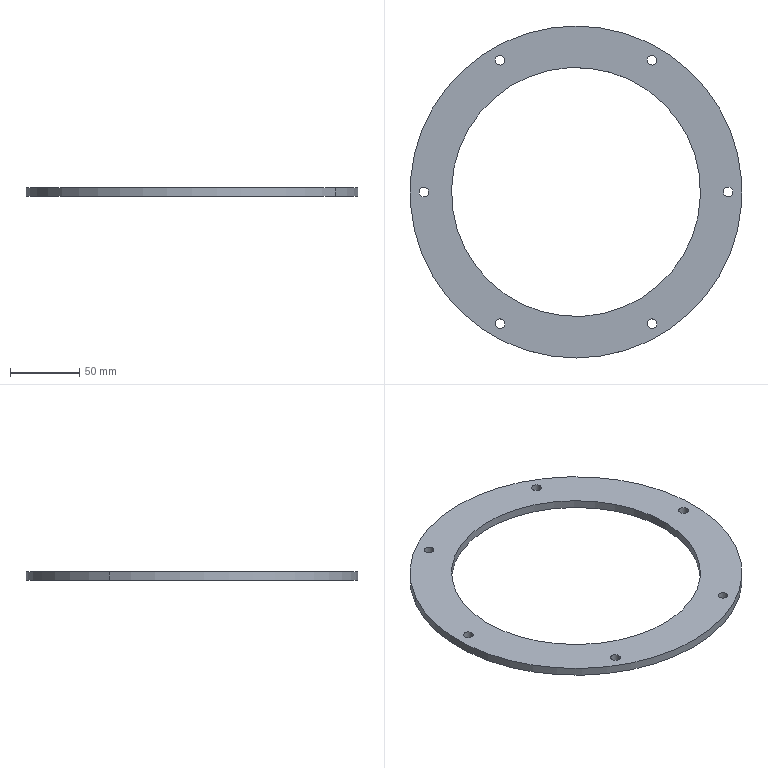Component | SolidWorks | YC1-250-02-03FrontDriveBearingSeatAssembly-1_YC1-250-02-23FrontDriveBearingSeatGland-1 | 1 solid | 18 faces | box 240 x 240 x 6 mm | volume 117367 mm3 | cylinder 16 | plane 2 | commonest cylinder face diameters 7 x12 180 x2 240 x2 | material Plain Carbon Steel
STEP:
#1=CARTESIAN_POINT('',(3.069,106.063,-17.48));
#2=VERTEX_POINT('',#1);
#3=CARTESIAN_POINT('',(-3.069,109.606,-17.48));
#4=VERTEX_POINT('',#3);
#5=CARTESIAN_POINT('',(0.,107.835,-17.48));
#6=DIRECTION('',(0.,0.,-1.));
#7=DIRECTION('',(-0.866,0.5,0.));
#8=AXIS2_PLACEMENT_3D('',#5,#6,#7);
#9=CIRCLE('',#8,3.543);
#10=EDGE_CURVE('',#2,#4,#9,.T.);
#11=ORIENTED_EDGE('',*,*,#10,.F.);
#12=CARTESIAN_POINT('',(3.069,106.063,-17.717));
#13=VERTEX_POINT('',#12);
#14=CARTESIAN_POINT('',(3.069,106.063,-17.48));
#15=DIRECTION('',(0.,0.,-1.));
#16=VECTOR('',#15,39.37);
#17=LINE('',#14,#16);
#18=EDGE_CURVE('',#2,#13,#17,.T.);
#19=ORIENTED_EDGE('',*,*,#18,.T.);
#20=CARTESIAN_POINT('',(-3.069,109.606,-17.717));
#21=VERTEX_POINT('',#20);
#22=CARTESIAN_POINT('',(0.,107.835,-17.717));
#23=DIRECTION('',(0.,0.,-1.));
#24=DIRECTION('',(-0.866,0.5,0.));
#25=AXIS2_PLACEMENT_3D('',#22,#23,#24);
#26=CIRCLE('',#25,3.543);
#27=EDGE_CURVE('',#13,#21,#26,.T.);
#28=ORIENTED_EDGE('',*,*,#27,.T.);
#29=CARTESIAN_POINT('',(-3.069,109.606,-17.48));
#30=DIRECTION('',(0.,0.,-1.));
#31=VECTOR('',#30,39.37);
#32=LINE('',#29,#31);
#33=EDGE_CURVE('',#4,#21,#32,.T.);
#34=ORIENTED_EDGE('',*,*,#33,.F.);
#35=EDGE_LOOP('',(#11,#19,#28,#34));
#36=FACE_OUTER_BOUND('',#35,.T.);
#37=CARTESIAN_POINT('',(0.,107.835,-17.48));
#38=DIRECTION('',(0.,0.,-1.));
#39=DIRECTION('',(-0.866,0.5,0.));
#40=AXIS2_PLACEMENT_3D('',#37,#38,#39);
#41=CYLINDRICAL_SURFACE('',#40,3.543);
#42=ADVANCED_FACE('',(#36),#41,.F.);
#43=CARTESIAN_POINT('',(-4.091,110.197,-17.48));
#44=VERTEX_POINT('',#43);
#45=CARTESIAN_POINT('',(4.091,105.472,-17.48));
#46=VERTEX_POINT('',#45);
#47=CARTESIAN_POINT('',(0.,107.835,-17.48));
#48=DIRECTION('',(0.,0.,-1.));
#49=DIRECTION('',(-0.866,0.5,0.));
#50=AXIS2_PLACEMENT_3D('',#47,#48,#49);
#51=CIRCLE('',#50,4.724);
#52=EDGE_CURVE('',#44,#46,#51,.T.);
#53=ORIENTED_EDGE('',*,*,#52,.T.);
#54=CARTESIAN_POINT('',(4.091,105.472,-17.717));
#55=VERTEX_POINT('',#54);
#56=CARTESIAN_POINT('',(4.091,105.472,-17.48));
#57=DIRECTION('',(0.,0.,-1.));
#58=VECTOR('',#57,39.37);
#59=LINE('',#56,#58);
#60=EDGE_CURVE('',#46,#55,#59,.T.);
#61=ORIENTED_EDGE('',*,*,#60,.T.);
#62=CARTESIAN_POINT('',(-4.091,110.197,-17.717));
#63=VERTEX_POINT('',#62);
#64=CARTESIAN_POINT('',(0.,107.835,-17.717));
#65=DIRECTION('',(0.,0.,1.));
#66=DIRECTION('',(-0.866,0.5,0.));
#67=AXIS2_PLACEMENT_3D('',#64,#65,#66);
#68=CIRCLE('',#67,4.724);
#69=EDGE_CURVE('',#55,#63,#68,.T.);
#70=ORIENTED_EDGE('',*,*,#69,.T.);
#71=CARTESIAN_POINT('',(-4.091,110.197,-17.48));
#72=DIRECTION('',(0.,0.,-1.));
#73=VECTOR('',#72,39.37);
#74=LINE('',#71,#73);
#75=EDGE_CURVE('',#44,#63,#74,.T.);
#76=ORIENTED_EDGE('',*,*,#75,.F.);
#77=EDGE_LOOP('',(#53,#61,#70,#76));
#78=FACE_OUTER_BOUND('',#77,.T.);
#79=CARTESIAN_POINT('',(0.,107.835,-17.48));
#80=DIRECTION('',(0.,0.,-1.));
#81=DIRECTION('',(-0.866,0.5,0.));
#82=AXIS2_PLACEMENT_3D('',#79,#80,#81);
#83=CYLINDRICAL_SURFACE('',#82,4.724);
#84=ADVANCED_FACE('',(#78),#83,.T.);
#85=CARTESIAN_POINT('',(-2.046,111.516,-17.717));
#86=VERTEX_POINT('',#85);
#87=CARTESIAN_POINT('',(-2.285,111.654,-17.717));
#88=VERTEX_POINT('',#87);
#89=CARTESIAN_POINT('',(-2.165,111.585,-17.717));
#90=DIRECTION('',(0.,0.,-1.));
#91=DIRECTION('',(0.866,-0.5,0.));
#92=AXIS2_PLACEMENT_3D('',#89,#90,#91);
#93=CIRCLE('',#92,0.1378);
#94=EDGE_CURVE('',#86,#88,#93,.T.);
#95=ORIENTED_EDGE('',*,*,#94,.T.);
#96=CARTESIAN_POINT('',(-2.285,111.654,-17.48));
#97=VERTEX_POINT('',#96);
#98=CARTESIAN_POINT('',(-2.285,111.654,-17.48));
#99=DIRECTION('',(0.,0.,1.));
#100=VECTOR('',#99,39.37);
#101=LINE('',#98,#100);
#102=EDGE_CURVE('',#88,#97,#101,.T.);
#103=ORIENTED_EDGE('',*,*,#102,.T.);
#104=CARTESIAN_POINT('',(-2.046,111.516,-17.48));
#105=VERTEX_POINT('',#104);
#106=CARTESIAN_POINT('',(-2.165,111.585,-17.48));
#107=DIRECTION('',(0.,0.,-1.));
#108=DIRECTION('',(0.866,-0.5,0.));
#109=AXIS2_PLACEMENT_3D('',#106,#107,#108);
#110=CIRCLE('',#109,0.1378);
#111=EDGE_CURVE('',#105,#97,#110,.T.);
#112=ORIENTED_EDGE('',*,*,#111,.F.);
#113=CARTESIAN_POINT('',(-2.046,111.516,-17.48));
#114=DIRECTION('',(0.,0.,1.));
#115=VECTOR('',#114,39.37);
#116=LINE('',#113,#115);
#117=EDGE_CURVE('',#86,#105,#116,.T.);
#118=ORIENTED_EDGE('',*,*,#117,.F.);
#119=EDGE_LOOP('',(#95,#103,#112,#118));
#120=FACE_OUTER_BOUND('',#119,.T.);
#121=CARTESIAN_POINT('',(-2.165,111.585,-17.48));
#122=DIRECTION('',(0.,0.,1.));
#123=DIRECTION('',(0.866,-0.5,0.));
#124=AXIS2_PLACEMENT_3D('',#121,#122,#123);
#125=CYLINDRICAL_SURFACE('',#124,0.1378);
#126=ADVANCED_FACE('',(#120),#125,.F.);
#127=CARTESIAN_POINT('',(-4.211,107.766,-17.717));
#128=VERTEX_POINT('',#127);
#129=CARTESIAN_POINT('',(-4.45,107.904,-17.717));
#130=VERTEX_POINT('',#129);
#131=CARTESIAN_POINT('',(-4.331,107.835,-17.717));
#132=DIRECTION('',(0.,0.,-1.));
#133=DIRECTION('',(0.866,-0.5,0.));
#134=AXIS2_PLACEMENT_3D('',#131,#132,#133);
#135=CIRCLE('',#134,0.1378);
#136=EDGE_CURVE('',#128,#130,#135,.T.);
#137=ORIENTED_EDGE('',*,*,#136,.T.);
#138=CARTESIAN_POINT('',(-4.45,107.904,-17.48));
#139=VERTEX_POINT('',#138);
#140=CARTESIAN_POINT('',(-4.45,107.904,-17.48));
#141=DIRECTION('',(0.,0.,1.));
#142=VECTOR('',#141,39.37);
#143=LINE('',#140,#142);
#144=EDGE_CURVE('',#130,#139,#143,.T.);
#145=ORIENTED_EDGE('',*,*,#144,.T.);
#146=CARTESIAN_POINT('',(-4.211,107.766,-17.48));
#147=VERTEX_POINT('',#146);
#148=CARTESIAN_POINT('',(-4.331,107.835,-17.48));
#149=DIRECTION('',(0.,0.,-1.));
#150=DIRECTION('',(0.866,-0.5,0.));
#151=AXIS2_PLACEMENT_3D('',#148,#149,#150);
#152=CIRCLE('',#151,0.1378);
#153=EDGE_CURVE('',#147,#139,#152,.T.);
#154=ORIENTED_EDGE('',*,*,#153,.F.);
#155=CARTESIAN_POINT('',(-4.211,107.766,-17.48));
#156=DIRECTION('',(0.,0.,1.));
#157=VECTOR('',#156,39.37);
#158=LINE('',#155,#157);
#159=EDGE_CURVE('',#128,#147,#158,.T.);
#160=ORIENTED_EDGE('',*,*,#159,.F.);
#161=EDGE_LOOP('',(#137,#145,#154,#160));
#162=FACE_OUTER_BOUND('',#161,.T.);
#163=CARTESIAN_POINT('',(-4.331,107.835,-17.48));
#164=DIRECTION('',(0.,0.,1.));
#165=DIRECTION('',(0.866,-0.5,0.));
#166=AXIS2_PLACEMENT_3D('',#163,#164,#165);
#167=CYLINDRICAL_SURFACE('',#166,0.1378);
#168=ADVANCED_FACE('',(#162),#167,.F.);
#169=CARTESIAN_POINT('',(-2.046,104.015,-17.717));
#170=VERTEX_POINT('',#169);
#171=CARTESIAN_POINT('',(-2.285,104.153,-17.717));
#172=VERTEX_POINT('',#171);
#173=CARTESIAN_POINT('',(-2.165,104.084,-17.717));
#174=DIRECTION('',(0.,0.,-1.));
#175=DIRECTION('',(0.866,-0.5,0.));
#176=AXIS2_PLACEMENT_3D('',#173,#174,#175);
#177=CIRCLE('',#176,0.1378);
#178=EDGE_CURVE('',#170,#172,#177,.T.);
#179=ORIENTED_EDGE('',*,*,#178,.T.);
#180=CARTESIAN_POINT('',(-2.285,104.153,-17.48));
#181=VERTEX_POINT('',#180);
#182=CARTESIAN_POINT('',(-2.285,104.153,-17.48));
#183=DIRECTION('',(0.,0.,1.));
#184=VECTOR('',#183,39.37);
#185=LINE('',#182,#184);
#186=EDGE_CURVE('',#172,#181,#185,.T.);
#187=ORIENTED_EDGE('',*,*,#186,.T.);
#188=CARTESIAN_POINT('',(-2.046,104.015,-17.48));
#189=VERTEX_POINT('',#188);
#190=CARTESIAN_POINT('',(-2.165,104.084,-17.48));
#191=DIRECTION('',(0.,0.,-1.));
#192=DIRECTION('',(0.866,-0.5,0.));
#193=AXIS2_PLACEMENT_3D('',#190,#191,#192);
#194=CIRCLE('',#193,0.1378);
#195=EDGE_CURVE('',#189,#181,#194,.T.);
#196=ORIENTED_EDGE('',*,*,#195,.F.);
#197=CARTESIAN_POINT('',(-2.046,104.015,-17.48));
#198=DIRECTION('',(0.,0.,1.));
#199=VECTOR('',#198,39.37);
#200=LINE('',#197,#199);
#201=EDGE_CURVE('',#170,#189,#200,.T.);
#202=ORIENTED_EDGE('',*,*,#201,.F.);
#203=EDGE_LOOP('',(#179,#187,#196,#202));
#204=FACE_OUTER_BOUND('',#203,.T.);
#205=CARTESIAN_POINT('',(-2.165,104.084,-17.48));
#206=DIRECTION('',(0.,0.,1.));
#207=DIRECTION('',(0.866,-0.5,0.));
#208=AXIS2_PLACEMENT_3D('',#205,#206,#207);
#209=CYLINDRICAL_SURFACE('',#208,0.1378);
#210=ADVANCED_FACE('',(#204),#209,.F.);
#211=CARTESIAN_POINT('',(2.285,104.015,-17.717));
#212=VERTEX_POINT('',#211);
#213=CARTESIAN_POINT('',(2.046,104.153,-17.717));
#214=VERTEX_POINT('',#213);
#215=CARTESIAN_POINT('',(2.165,104.084,-17.717));
#216=DIRECTION('',(0.,0.,-1.));
#217=DIRECTION('',(0.866,-0.5,0.));
#218=AXIS2_PLACEMENT_3D('',#215,#216,#217);
#219=CIRCLE('',#218,0.1378);
#220=EDGE_CURVE('',#212,#214,#219,.T.);
#221=ORIENTED_EDGE('',*,*,#220,.T.);
#222=CARTESIAN_POINT('',(2.046,104.153,-17.48));
#223=VERTEX_POINT('',#222);
#224=CARTESIAN_POINT('',(2.046,104.153,-17.48));
#225=DIRECTION('',(0.,0.,1.));
#226=VECTOR('',#225,39.37);
#227=LINE('',#224,#226);
#228=EDGE_CURVE('',#214,#223,#227,.T.);
#229=ORIENTED_EDGE('',*,*,#228,.T.);
#230=CARTESIAN_POINT('',(2.285,104.015,-17.48));
#231=VERTEX_POINT('',#230);
#232=CARTESIAN_POINT('',(2.165,104.084,-17.48));
#233=DIRECTION('',(0.,0.,-1.));
#234=DIRECTION('',(0.866,-0.5,0.));
#235=AXIS2_PLACEMENT_3D('',#232,#233,#234);
#236=CIRCLE('',#235,0.1378);
#237=EDGE_CURVE('',#231,#223,#236,.T.);
#238=ORIENTED_EDGE('',*,*,#237,.F.);
#239=CARTESIAN_POINT('',(2.285,104.015,-17.48));
#240=DIRECTION('',(0.,0.,1.));
#241=VECTOR('',#240,39.37);
#242=LINE('',#239,#241);
#243=EDGE_CURVE('',#212,#231,#242,.T.);
#244=ORIENTED_EDGE('',*,*,#243,.F.);
#245=EDGE_LOOP('',(#221,#229,#238,#244));
#246=FACE_OUTER_BOUND('',#245,.T.);
#247=CARTESIAN_POINT('',(2.165,104.084,-17.48));
#248=DIRECTION('',(0.,0.,1.));
#249=DIRECTION('',(0.866,-0.5,0.));
#250=AXIS2_PLACEMENT_3D('',#247,#248,#249);
#251=CYLINDRICAL_SURFACE('',#250,0.1378);
#252=ADVANCED_FACE('',(#246),#251,.F.);
#253=CARTESIAN_POINT('',(4.45,107.766,-17.717));
#254=VERTEX_POINT('',#253);
#255=CARTESIAN_POINT('',(4.211,107.904,-17.717));
#256=VERTEX_POINT('',#255);
#257=CARTESIAN_POINT('',(4.331,107.835,-17.717));
#258=DIRECTION('',(0.,0.,-1.));
#259=DIRECTION('',(0.866,-0.5,0.));
#260=AXIS2_PLACEMENT_3D('',#257,#258,#259);
#261=CIRCLE('',#260,0.1378);
#262=EDGE_CURVE('',#254,#256,#261,.T.);
#263=ORIENTED_EDGE('',*,*,#262,.T.);
#264=CARTESIAN_POINT('',(4.211,107.904,-17.48));
#265=VERTEX_POINT('',#264);
#266=CARTESIAN_POINT('',(4.211,107.904,-17.48));
#267=DIRECTION('',(0.,0.,1.));
#268=VECTOR('',#267,39.37);
#269=LINE('',#266,#268);
#270=EDGE_CURVE('',#256,#265,#269,.T.);
#271=ORIENTED_EDGE('',*,*,#270,.T.);
#272=CARTESIAN_POINT('',(4.45,107.766,-17.48));
#273=VERTEX_POINT('',#272);
#274=CARTESIAN_POINT('',(4.331,107.835,-17.48));
#275=DIRECTION('',(0.,0.,-1.));
#276=DIRECTION('',(0.866,-0.5,0.));
#277=AXIS2_PLACEMENT_3D('',#274,#275,#276);
#278=CIRCLE('',#277,0.1378);
#279=EDGE_CURVE('',#273,#265,#278,.T.);
#280=ORIENTED_EDGE('',*,*,#279,.F.);
#281=CARTESIAN_POINT('',(4.45,107.766,-17.48));
#282=DIRECTION('',(0.,0.,1.));
#283=VECTOR('',#282,39.37);
#284=LINE('',#281,#283);
#285=EDGE_CURVE('',#254,#273,#284,.T.);
#286=ORIENTED_EDGE('',*,*,#285,.F.);
#287=EDGE_LOOP('',(#263,#271,#280,#286));
#288=FACE_OUTER_BOUND('',#287,.T.);
#289=CARTESIAN_POINT('',(4.331,107.835,-17.48));
#290=DIRECTION('',(0.,0.,1.));
#291=DIRECTION('',(0.866,-0.5,0.));
#292=AXIS2_PLACEMENT_3D('',#289,#290,#291);
#293=CYLINDRICAL_SURFACE('',#292,0.1378);
#294=ADVANCED_FACE('',(#288),#293,.F.);
#295=CARTESIAN_POINT('',(2.285,111.516,-17.717));
#296=VERTEX_POINT('',#295);
#297=CARTESIAN_POINT('',(2.046,111.654,-17.717));
#298=VERTEX_POINT('',#297);
#299=CARTESIAN_POINT('',(2.165,111.585,-17.717));
#300=DIRECTION('',(0.,0.,-1.));
#301=DIRECTION('',(0.866,-0.5,0.));
#302=AXIS2_PLACEMENT_3D('',#299,#300,#301);
#303=CIRCLE('',#302,0.1378);
#304=EDGE_CURVE('',#296,#298,#303,.T.);
#305=ORIENTED_EDGE('',*,*,#304,.T.);
#306=CARTESIAN_POINT('',(2.046,111.654,-17.48));
#307=VERTEX_POINT('',#306);
#308=CARTESIAN_POINT('',(2.046,111.654,-17.48));
#309=DIRECTION('',(0.,0.,1.));
#310=VECTOR('',#309,39.37);
#311=LINE('',#308,#310);
#312=EDGE_CURVE('',#298,#307,#311,.T.);
#313=ORIENTED_EDGE('',*,*,#312,.T.);
#314=CARTESIAN_POINT('',(2.285,111.516,-17.48));
#315=VERTEX_POINT('',#314);
#316=CARTESIAN_POINT('',(2.165,111.585,-17.48));
#317=DIRECTION('',(0.,0.,-1.));
#318=DIRECTION('',(0.866,-0.5,0.));
#319=AXIS2_PLACEMENT_3D('',#316,#317,#318);
#320=CIRCLE('',#319,0.1378);
#321=EDGE_CURVE('',#315,#307,#320,.T.);
#322=ORIENTED_EDGE('',*,*,#321,.F.);
#323=CARTESIAN_POINT('',(2.285,111.516,-17.48));
#324=DIRECTION('',(0.,0.,1.));
#325=VECTOR('',#324,39.37);
#326=LINE('',#323,#325);
#327=EDGE_CURVE('',#296,#315,#326,.T.);
#328=ORIENTED_EDGE('',*,*,#327,.F.);
#329=EDGE_LOOP('',(#305,#313,#322,#328));
#330=FACE_OUTER_BOUND('',#329,.T.);
#331=CARTESIAN_POINT('',(2.165,111.585,-17.48));
#332=DIRECTION('',(0.,0.,1.));
#333=DIRECTION('',(0.866,-0.5,0.));
#334=AXIS2_PLACEMENT_3D('',#331,#332,#333);
#335=CYLINDRICAL_SURFACE('',#334,0.1378);
#336=ADVANCED_FACE('',(#330),#335,.F.);
#337=CARTESIAN_POINT('',(0.,107.835,-17.717));
#338=DIRECTION('',(0.,0.,-1.));
#339=DIRECTION('',(-0.866,0.5,0.));
#340=AXIS2_PLACEMENT_3D('',#337,#338,#339);
#341=CIRCLE('',#340,3.543);
#342=EDGE_CURVE('',#21,#13,#341,.T.);
#343=ORIENTED_EDGE('',*,*,#342,.F.);
#344=ORIENTED_EDGE('',*,*,#27,.F.);
#345=EDGE_LOOP('',(#343,#344));
#346=FACE_BOUND('',#345,.T.);
#347=CARTESIAN_POINT('',(0.,107.835,-17.717));
#348=DIRECTION('',(0.,0.,1.));
#349=DIRECTION('',(-0.866,0.5,0.));
#350=AXIS2_PLACEMENT_3D('',#347,#348,#349);
#351=CIRCLE('',#350,4.724);
#352=EDGE_CURVE('',#63,#55,#351,.T.);
#353=ORIENTED_EDGE('',*,*,#352,.F.);
#354=ORIENTED_EDGE('',*,*,#69,.F.);
#355=EDGE_LOOP('',(#353,#354));
#356=FACE_OUTER_BOUND('',#355,.T.);
#357=ORIENTED_EDGE('',*,*,#94,.F.);
#358=CARTESIAN_POINT('',(-2.165,111.585,-17.717));
#359=DIRECTION('',(0.,0.,-1.));
#360=DIRECTION('',(0.866,-0.5,0.));
#361=AXIS2_PLACEMENT_3D('',#358,#359,#360);
#362=CIRCLE('',#361,0.1378);
#363=EDGE_CURVE('',#88,#86,#362,.T.);
#364=ORIENTED_EDGE('',*,*,#363,.F.);
#365=EDGE_LOOP('',(#357,#364));
#366=FACE_BOUND('',#365,.T.);
#367=ORIENTED_EDGE('',*,*,#136,.F.);
#368=CARTESIAN_POINT('',(-4.331,107.835,-17.717));
#369=DIRECTION('',(0.,0.,-1.));
#370=DIRECTION('',(0.866,-0.5,0.));
#371=AXIS2_PLACEMENT_3D('',#368,#369,#370);
#372=CIRCLE('',#371,0.1378);
#373=EDGE_CURVE('',#130,#128,#372,.T.);
#374=ORIENTED_EDGE('',*,*,#373,.F.);
#375=EDGE_LOOP('',(#367,#374));
#376=FACE_BOUND('',#375,.T.);
#377=ORIENTED_EDGE('',*,*,#178,.F.);
#378=CARTESIAN_POINT('',(-2.165,104.084,-17.717));
#379=DIRECTION('',(0.,0.,-1.));
#380=DIRECTION('',(0.866,-0.5,0.));
#381=AXIS2_PLACEMENT_3D('',#378,#379,#380);
#382=CIRCLE('',#381,0.1378);
#383=EDGE_CURVE('',#172,#170,#382,.T.);
#384=ORIENTED_EDGE('',*,*,#383,.F.);
#385=EDGE_LOOP('',(#377,#384));
#386=FACE_BOUND('',#385,.T.);
#387=ORIENTED_EDGE('',*,*,#220,.F.);
#388=CARTESIAN_POINT('',(2.165,104.084,-17.717));
#389=DIRECTION('',(0.,0.,-1.));
#390=DIRECTION('',(0.866,-0.5,0.));
#391=AXIS2_PLACEMENT_3D('',#388,#389,#390);
#392=CIRCLE('',#391,0.1378);
#393=EDGE_CURVE('',#214,#212,#392,.T.);
#394=ORIENTED_EDGE('',*,*,#393,.F.);
#395=EDGE_LOOP('',(#387,#394));
#396=FACE_BOUND('',#395,.T.);
#397=ORIENTED_EDGE('',*,*,#262,.F.);
#398=CARTESIAN_POINT('',(4.331,107.835,-17.717));
#399=DIRECTION('',(0.,0.,-1.));
#400=DIRECTION('',(0.866,-0.5,0.));
#401=AXIS2_PLACEMENT_3D('',#398,#399,#400);
#402=CIRCLE('',#401,0.1378);
#403=EDGE_CURVE('',#256,#254,#402,.T.);
#404=ORIENTED_EDGE('',*,*,#403,.F.);
#405=EDGE_LOOP('',(#397,#404));
#406=FACE_BOUND('',#405,.T.);
#407=ORIENTED_EDGE('',*,*,#304,.F.);
#408=CARTESIAN_POINT('',(2.165,111.585,-17.717));
#409=DIRECTION('',(0.,0.,-1.));
#410=DIRECTION('',(0.866,-0.5,0.));
#411=AXIS2_PLACEMENT_3D('',#408,#409,#410);
#412=CIRCLE('',#411,0.1378);
#413=EDGE_CURVE('',#298,#296,#412,.T.);
#414=ORIENTED_EDGE('',*,*,#413,.F.);
#415=EDGE_LOOP('',(#407,#414));
#416=FACE_BOUND('',#415,.T.);
#417=CARTESIAN_POINT('',(0.,107.835,-17.717));
#418=DIRECTION('',(0.,0.,1.));
#419=DIRECTION('',(0.866,-0.5,0.));
#420=AXIS2_PLACEMENT_3D('',#417,#418,#419);
#421=PLANE('',#420);
#422=ADVANCED_FACE('',(#346,#356,#366,#376,#386,#396,#406,#416),#421,.F.);
#423=ORIENTED_EDGE('',*,*,#18,.F.);
#424=CARTESIAN_POINT('',(0.,107.835,-17.48));
#425=DIRECTION('',(0.,0.,-1.));
#426=DIRECTION('',(-0.866,0.5,0.));
#427=AXIS2_PLACEMENT_3D('',#424,#425,#426);
#428=CIRCLE('',#427,3.543);
#429=EDGE_CURVE('',#4,#2,#428,.T.);
#430=ORIENTED_EDGE('',*,*,#429,.F.);
#431=ORIENTED_EDGE('',*,*,#33,.T.);
#432=ORIENTED_EDGE('',*,*,#342,.T.);
#433=EDGE_LOOP('',(#423,#430,#431,#432));
#434=FACE_OUTER_BOUND('',#433,.T.);
#435=CARTESIAN_POINT('',(0.,107.835,-17.48));
#436=DIRECTION('',(0.,0.,-1.));
#437=DIRECTION('',(-0.866,0.5,0.));
#438=AXIS2_PLACEMENT_3D('',#435,#436,#437);
#439=CYLINDRICAL_SURFACE('',#438,3.543);
#440=ADVANCED_FACE('',(#434),#439,.F.);
#441=ORIENTED_EDGE('',*,*,#60,.F.);
#442=CARTESIAN_POINT('',(0.,107.835,-17.48));
#443=DIRECTION('',(0.,0.,-1.));
#444=DIRECTION('',(-0.866,0.5,0.));
#445=AXIS2_PLACEMENT_3D('',#442,#443,#444);
#446=CIRCLE('',#445,4.724);
#447=EDGE_CURVE('',#46,#44,#446,.T.);
#448=ORIENTED_EDGE('',*,*,#447,.T.);
#449=ORIENTED_EDGE('',*,*,#75,.T.);
#450=ORIENTED_EDGE('',*,*,#352,.T.);
#451=EDGE_LOOP('',(#441,#448,#449,#450));
#452=FACE_OUTER_BOUND('',#451,.T.);
#453=CARTESIAN_POINT('',(0.,107.835,-17.48));
#454=DIRECTION('',(0.,0.,-1.));
#455=DIRECTION('',(-0.866,0.5,0.));
#456=AXIS2_PLACEMENT_3D('',#453,#454,#455);
#457=CYLINDRICAL_SURFACE('',#456,4.724);
#458=ADVANCED_FACE('',(#452),#457,.T.);
#459=ORIENTED_EDGE('',*,*,#102,.F.);
#460=ORIENTED_EDGE('',*,*,#363,.T.);
#461=ORIENTED_EDGE('',*,*,#117,.T.);
#462=CARTESIAN_POINT('',(-2.165,111.585,-17.48));
#463=DIRECTION('',(0.,0.,-1.));
#464=DIRECTION('',(0.866,-0.5,0.));
#465=AXIS2_PLACEMENT_3D('',#462,#463,#464);
#466=CIRCLE('',#465,0.1378);
#467=EDGE_CURVE('',#97,#105,#466,.T.);
#468=ORIENTED_EDGE('',*,*,#467,.F.);
#469=EDGE_LOOP('',(#459,#460,#461,#468));
#470=FACE_OUTER_BOUND('',#469,.T.);
#471=CARTESIAN_POINT('',(-2.165,111.585,-17.48));
#472=DIRECTION('',(0.,0.,1.));
#473=DIRECTION('',(0.866,-0.5,0.));
#474=AXIS2_PLACEMENT_3D('',#471,#472,#473);
#475=CYLINDRICAL_SURFACE('',#474,0.1378);
#476=ADVANCED_FACE('',(#470),#475,.F.);
#477=ORIENTED_EDGE('',*,*,#144,.F.);
#478=ORIENTED_EDGE('',*,*,#373,.T.);
#479=ORIENTED_EDGE('',*,*,#159,.T.);
#480=CARTESIAN_POINT('',(-4.331,107.835,-17.48));
#481=DIRECTION('',(0.,0.,-1.));
#482=DIRECTION('',(0.866,-0.5,0.));
#483=AXIS2_PLACEMENT_3D('',#480,#481,#482);
#484=CIRCLE('',#483,0.1378);
#485=EDGE_CURVE('',#139,#147,#484,.T.);
#486=ORIENTED_EDGE('',*,*,#485,.F.);
#487=EDGE_LOOP('',(#477,#478,#479,#486));
#488=FACE_OUTER_BOUND('',#487,.T.);
#489=CARTESIAN_POINT('',(-4.331,107.835,-17.48));
#490=DIRECTION('',(0.,0.,1.));
#491=DIRECTION('',(0.866,-0.5,0.));
#492=AXIS2_PLACEMENT_3D('',#489,#490,#491);
#493=CYLINDRICAL_SURFACE('',#492,0.1378);
#494=ADVANCED_FACE('',(#488),#493,.F.);
#495=ORIENTED_EDGE('',*,*,#186,.F.);
#496=ORIENTED_EDGE('',*,*,#383,.T.);
#497=ORIENTED_EDGE('',*,*,#201,.T.);
#498=CARTESIAN_POINT('',(-2.165,104.084,-17.48));
#499=DIRECTION('',(0.,0.,-1.));
#500=DIRECTION('',(0.866,-0.5,0.));
#501=AXIS2_PLACEMENT_3D('',#498,#499,#500);
#502=CIRCLE('',#501,0.1378);
#503=EDGE_CURVE('',#181,#189,#502,.T.);
#504=ORIENTED_EDGE('',*,*,#503,.F.);
#505=EDGE_LOOP('',(#495,#496,#497,#504));
#506=FACE_OUTER_BOUND('',#505,.T.);
#507=CARTESIAN_POINT('',(-2.165,104.084,-17.48));
#508=DIRECTION('',(0.,0.,1.));
#509=DIRECTION('',(0.866,-0.5,0.));
#510=AXIS2_PLACEMENT_3D('',#507,#508,#509);
#511=CYLINDRICAL_SURFACE('',#510,0.1378);
#512=ADVANCED_FACE('',(#506),#511,.F.);
#513=ORIENTED_EDGE('',*,*,#228,.F.);
#514=ORIENTED_EDGE('',*,*,#393,.T.);
#515=ORIENTED_EDGE('',*,*,#243,.T.);
#516=CARTESIAN_POINT('',(2.165,104.084,-17.48));
#517=DIRECTION('',(0.,0.,-1.));
#518=DIRECTION('',(0.866,-0.5,0.));
#519=AXIS2_PLACEMENT_3D('',#516,#517,#518);
#520=CIRCLE('',#519,0.1378);
#521=EDGE_CURVE('',#223,#231,#520,.T.);
#522=ORIENTED_EDGE('',*,*,#521,.F.);
#523=EDGE_LOOP('',(#513,#514,#515,#522));
#524=FACE_OUTER_BOUND('',#523,.T.);
#525=CARTESIAN_POINT('',(2.165,104.084,-17.48));
#526=DIRECTION('',(0.,0.,1.));
#527=DIRECTION('',(0.866,-0.5,0.));
#528=AXIS2_PLACEMENT_3D('',#525,#526,#527);
#529=CYLINDRICAL_SURFACE('',#528,0.1378);
#530=ADVANCED_FACE('',(#524),#529,.F.);
#531=ORIENTED_EDGE('',*,*,#270,.F.);
#532=ORIENTED_EDGE('',*,*,#403,.T.);
#533=ORIENTED_EDGE('',*,*,#285,.T.);
#534=CARTESIAN_POINT('',(4.331,107.835,-17.48));
#535=DIRECTION('',(0.,0.,-1.));
#536=DIRECTION('',(0.866,-0.5,0.));
#537=AXIS2_PLACEMENT_3D('',#534,#535,#536);
#538=CIRCLE('',#537,0.1378);
#539=EDGE_CURVE('',#265,#273,#538,.T.);
#540=ORIENTED_EDGE('',*,*,#539,.F.);
#541=EDGE_LOOP('',(#531,#532,#533,#540));
#542=FACE_OUTER_BOUND('',#541,.T.);
#543=CARTESIAN_POINT('',(4.331,107.835,-17.48));
#544=DIRECTION('',(0.,0.,1.));
#545=DIRECTION('',(0.866,-0.5,0.));
#546=AXIS2_PLACEMENT_3D('',#543,#544,#545);
#547=CYLINDRICAL_SURFACE('',#546,0.1378);
#548=ADVANCED_FACE('',(#542),#547,.F.);
#549=ORIENTED_EDGE('',*,*,#312,.F.);
#550=ORIENTED_EDGE('',*,*,#413,.T.);
#551=ORIENTED_EDGE('',*,*,#327,.T.);
#552=CARTESIAN_POINT('',(2.165,111.585,-17.48));
#553=DIRECTION('',(0.,0.,-1.));
#554=DIRECTION('',(0.866,-0.5,0.));
#555=AXIS2_PLACEMENT_3D('',#552,#553,#554);
#556=CIRCLE('',#555,0.1378);
#557=EDGE_CURVE('',#307,#315,#556,.T.);
#558=ORIENTED_EDGE('',*,*,#557,.F.);
#559=EDGE_LOOP('',(#549,#550,#551,#558));
#560=FACE_OUTER_BOUND('',#559,.T.);
#561=CARTESIAN_POINT('',(2.165,111.585,-17.48));
#562=DIRECTION('',(0.,0.,1.));
#563=DIRECTION('',(0.866,-0.5,0.));
#564=AXIS2_PLACEMENT_3D('',#561,#562,#563);
#565=CYLINDRICAL_SURFACE('',#564,0.1378);
#566=ADVANCED_FACE('',(#560),#565,.F.);
#567=ORIENTED_EDGE('',*,*,#429,.T.);
#568=ORIENTED_EDGE('',*,*,#10,.T.);
#569=EDGE_LOOP('',(#567,#568));
#570=FACE_BOUND('',#569,.T.);
#571=ORIENTED_EDGE('',*,*,#52,.F.);
#572=ORIENTED_EDGE('',*,*,#447,.F.);
#573=EDGE_LOOP('',(#571,#572));
#574=FACE_OUTER_BOUND('',#573,.T.);
#575=ORIENTED_EDGE('',*,*,#111,.T.);
#576=ORIENTED_EDGE('',*,*,#467,.T.);
#577=EDGE_LOOP('',(#575,#576));
#578=FACE_BOUND('',#577,.T.);
#579=ORIENTED_EDGE('',*,*,#153,.T.);
#580=ORIENTED_EDGE('',*,*,#485,.T.);
#581=EDGE_LOOP('',(#579,#580));
#582=FACE_BOUND('',#581,.T.);
#583=ORIENTED_EDGE('',*,*,#195,.T.);
#584=ORIENTED_EDGE('',*,*,#503,.T.);
#585=EDGE_LOOP('',(#583,#584));
#586=FACE_BOUND('',#585,.T.);
#587=ORIENTED_EDGE('',*,*,#237,.T.);
#588=ORIENTED_EDGE('',*,*,#521,.T.);
#589=EDGE_LOOP('',(#587,#588));
#590=FACE_BOUND('',#589,.T.);
#591=ORIENTED_EDGE('',*,*,#279,.T.);
#592=ORIENTED_EDGE('',*,*,#539,.T.);
#593=EDGE_LOOP('',(#591,#592));
#594=FACE_BOUND('',#593,.T.);
#595=ORIENTED_EDGE('',*,*,#321,.T.);
#596=ORIENTED_EDGE('',*,*,#557,.T.);
#597=EDGE_LOOP('',(#595,#596));
#598=FACE_BOUND('',#597,.T.);
#599=CARTESIAN_POINT('',(0.,107.835,-17.48));
#600=DIRECTION('',(0.,0.,1.));
#601=DIRECTION('',(0.866,-0.5,0.));
#602=AXIS2_PLACEMENT_3D('',#599,#600,#601);
#603=PLANE('',#602);
#604=ADVANCED_FACE('',(#570,#574,#578,#582,#586,#590,#594,#598),#603,.T.);
#605=CLOSED_SHELL('',(#42,#84,#126,#168,#210,#252,#294,#336,#422,#440,#458,#476,#494,#512,#530,#548,#566,#604));
#606=MANIFOLD_SOLID_BREP('',#605);
#607=CARTESIAN_POINT('',(0.,0.,0.));
#608=DIRECTION('',(0.,0.,1.));
#609=DIRECTION('',(1.,0.,0.));
#610=AXIS2_PLACEMENT_3D('',#607,#608,#609);
#611=(LENGTH_UNIT()NAMED_UNIT(*)SI_UNIT($,.METRE.));
#612=LENGTH_MEASURE_WITH_UNIT(LENGTH_MEASURE(0.0254),#611);
#613=DIMENSIONAL_EXPONENTS(1.,0.,0.,0.,0.,0.,0.);
#614=(CONVERSION_BASED_UNIT('',#612)LENGTH_UNIT()NAMED_UNIT(#613));
#615=UNCERTAINTY_MEASURE_WITH_UNIT(LENGTH_MEASURE(0.00001),#614,'','');
#616=(NAMED_UNIT(*)PLANE_ANGLE_UNIT()SI_UNIT($,.RADIAN.));
#617=(NAMED_UNIT(*)SI_UNIT($,.STERADIAN.)SOLID_ANGLE_UNIT());
#618=(GEOMETRIC_REPRESENTATION_CONTEXT(3)GLOBAL_UNCERTAINTY_ASSIGNED_CONTEXT((#615))GLOBAL_UNIT_ASSIGNED_CONTEXT((#614,#616,#617))REPRESENTATION_CONTEXT('',''));
#619=ADVANCED_BREP_SHAPE_REPRESENTATION('',(#606,#610),#618);
#620=COLOUR_RGB('',0.7922,0.8196,0.9333);
#621=FILL_AREA_STYLE_COLOUR('',#620);
#622=FILL_AREA_STYLE('',(#621));
#623=SURFACE_STYLE_FILL_AREA(#622);
#624=SURFACE_SIDE_STYLE('',(#623));
#625=SURFACE_STYLE_USAGE(.BOTH.,#624);
#626=PRESENTATION_STYLE_ASSIGNMENT((#625));
#627=STYLED_ITEM('',(#626),#606);
#628=PRESENTATION_LAYER_ASSIGNMENT('','',(#627));
#629=(LENGTH_UNIT()NAMED_UNIT(*)SI_UNIT($,.METRE.));
#630=LENGTH_MEASURE_WITH_UNIT(LENGTH_MEASURE(0.0254),#629);
#631=DIMENSIONAL_EXPONENTS(1.,0.,0.,0.,0.,0.,0.);
#632=(CONVERSION_BASED_UNIT('',#630)LENGTH_UNIT()NAMED_UNIT(#631));
#633=UNCERTAINTY_MEASURE_WITH_UNIT(LENGTH_MEASURE(0.00001),#632,'','');
#634=(NAMED_UNIT(*)PLANE_ANGLE_UNIT()SI_UNIT($,.RADIAN.));
#635=(NAMED_UNIT(*)SI_UNIT($,.STERADIAN.)SOLID_ANGLE_UNIT());
#636=(GEOMETRIC_REPRESENTATION_CONTEXT(3)GLOBAL_UNCERTAINTY_ASSIGNED_CONTEXT((#633))GLOBAL_UNIT_ASSIGNED_CONTEXT((#632,#634,#635))REPRESENTATION_CONTEXT('',''));
#637=MECHANICAL_DESIGN_GEOMETRIC_PRESENTATION_REPRESENTATION('',(#627),#636);